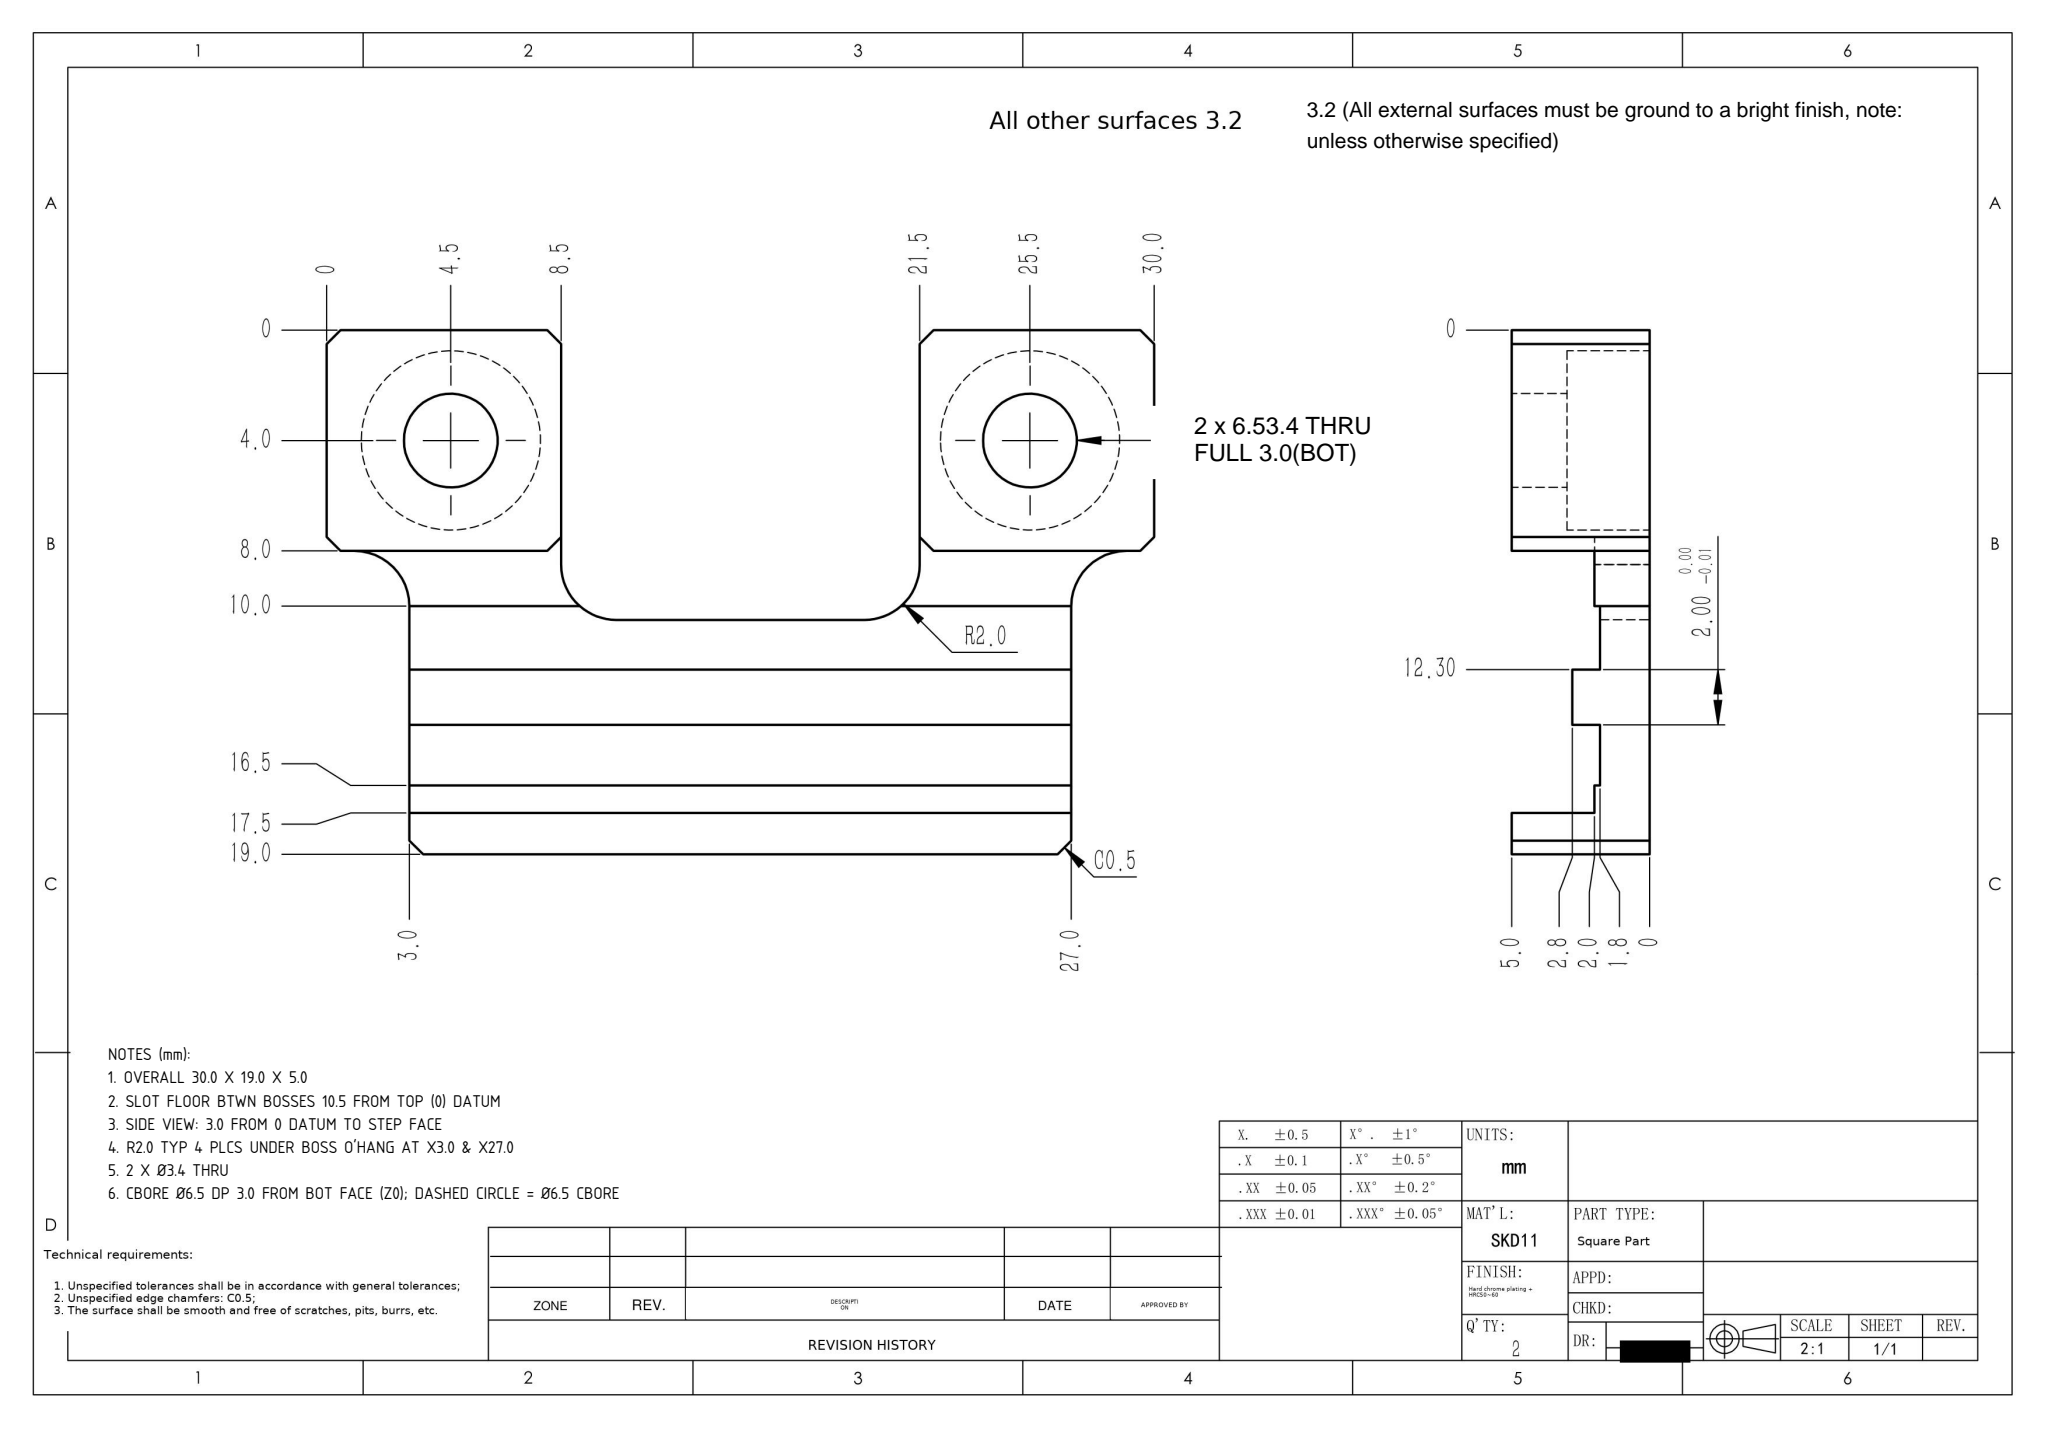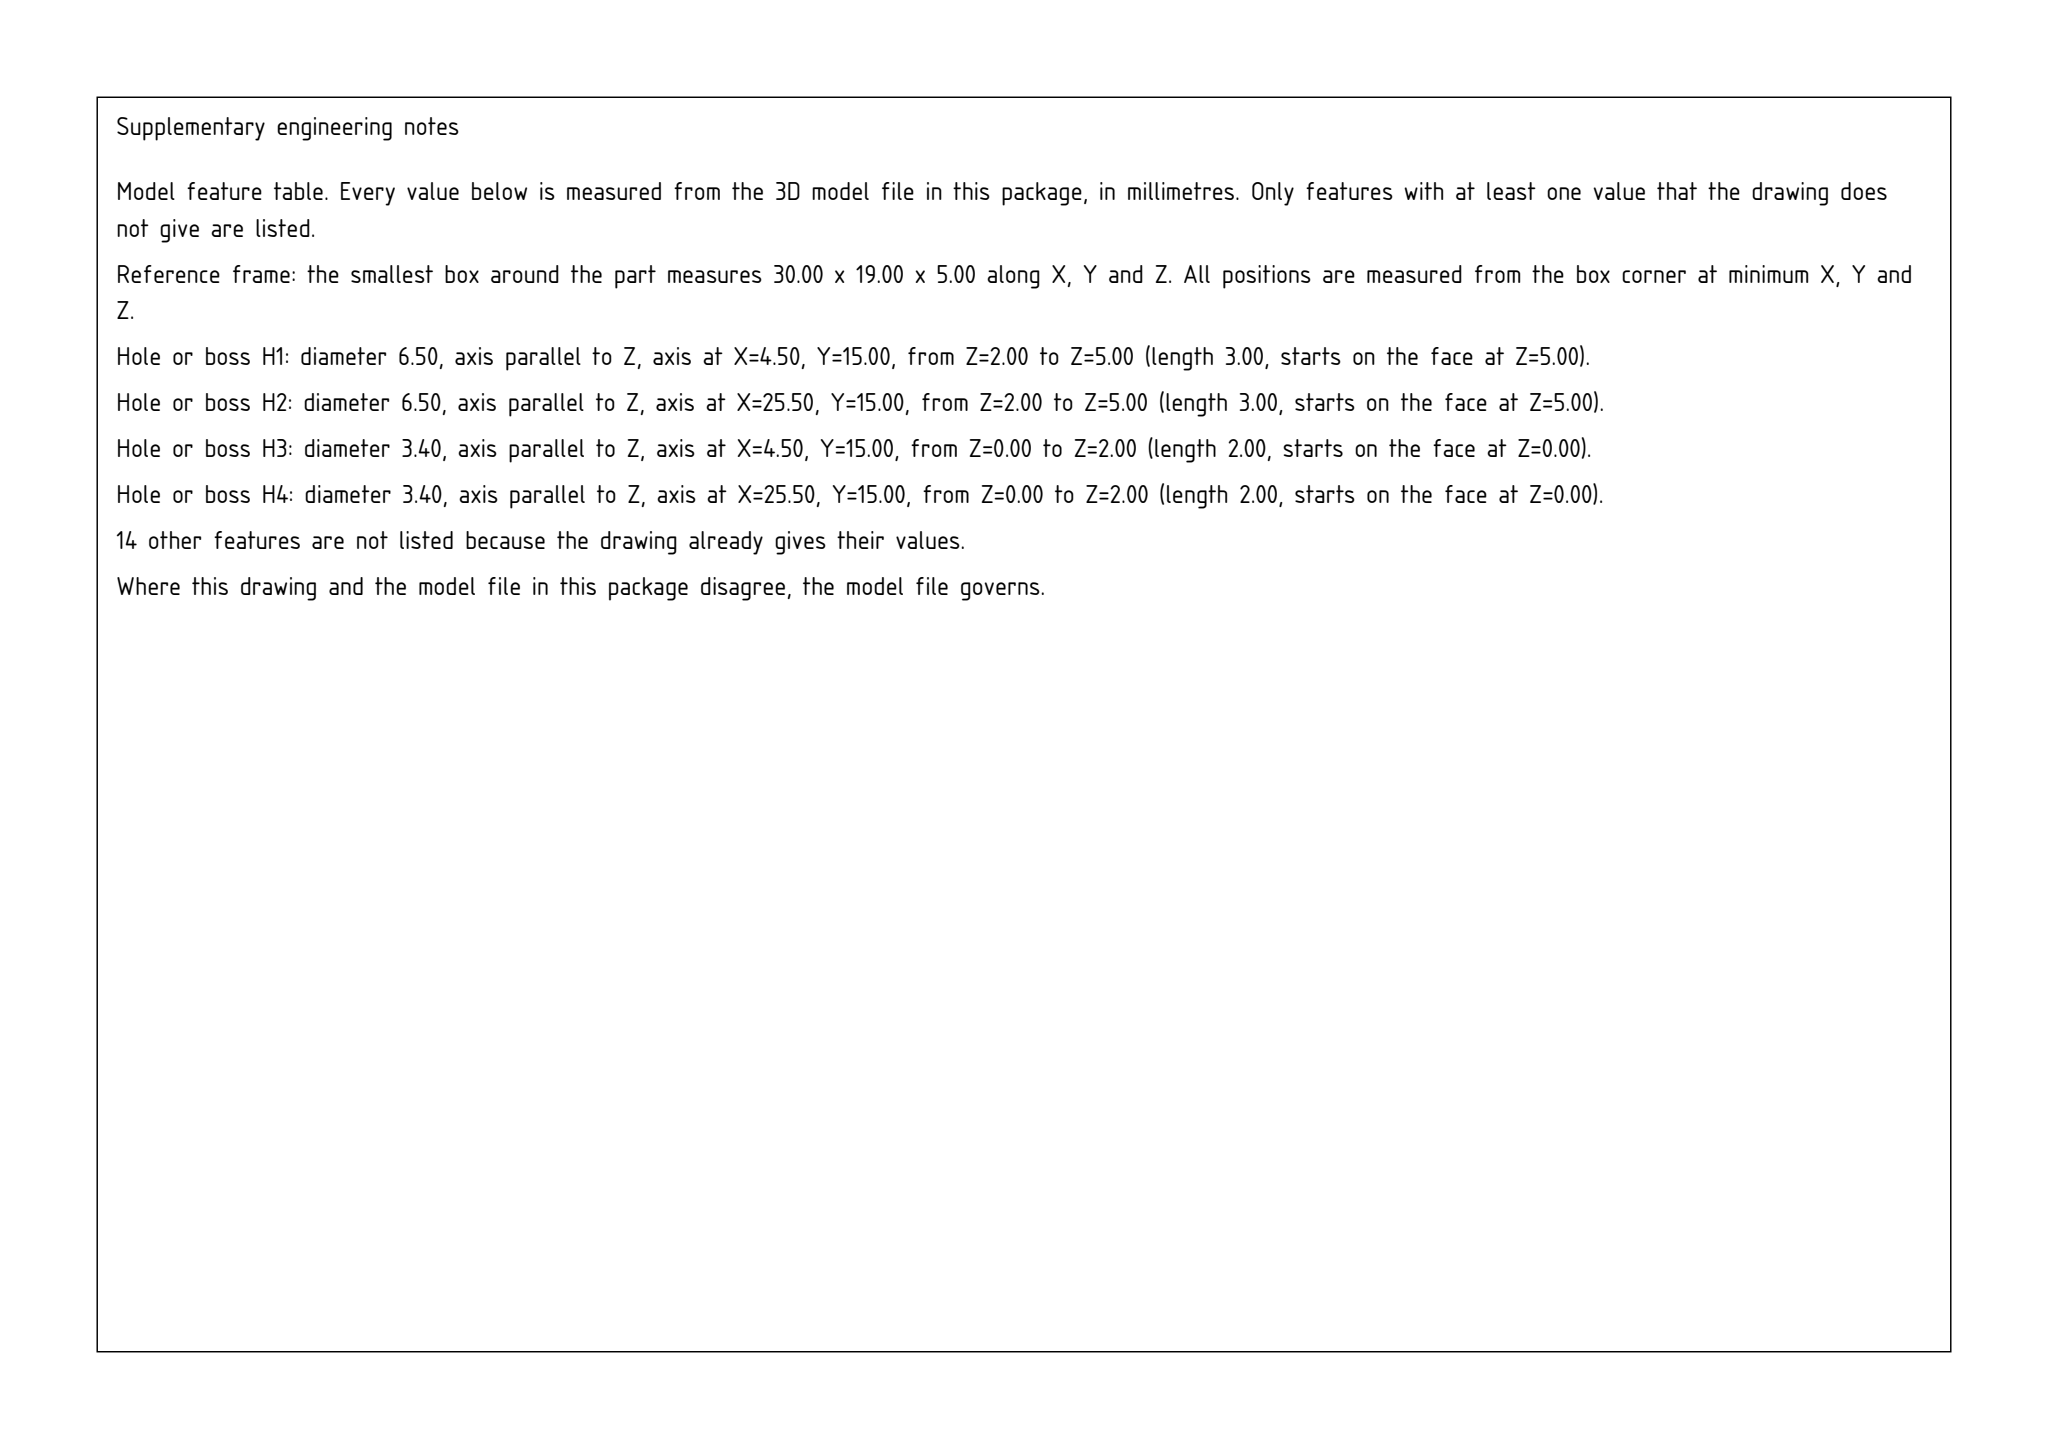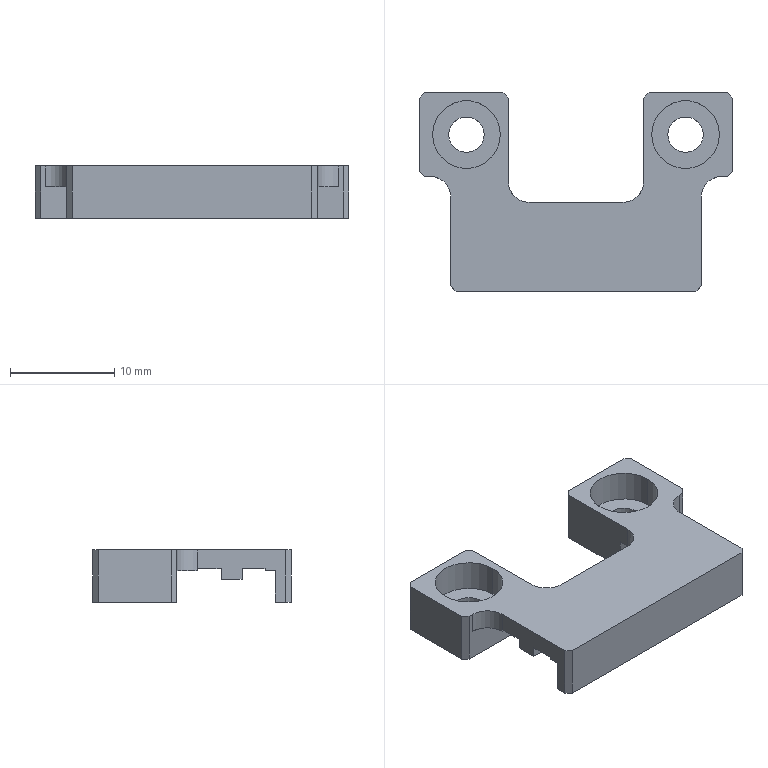Part | SolidWorks | mm | 1 solid | 52 faces | box 30 x 19 x 5 mm | volume 1035 mm3 | plane 40 | cylinder 12 | commonest cylinder face diameters 6.5 x4 3.4 x4 4 x4
Drawing notes:
OVERALL 30.0 X 19.0 X 5.0 | from the solid: bbox_xyz 30.0 x 19.0 x 5.0
SLOT FLOOR BTWN BOSSES 10.5 FROM TOP (0) DATUM | from the solid: Y-plane 8.5 in 19.0-tall bbox = 19.0-8.5 = 10.5 below top datum Y19.0
SIDE VIEW: 3.0 FROM 0 DATUM TO STEP FACE | from the solid: Z-plane 2.0 in 5.0 thk = 5.0-2.0 = 3.0 from side-view 0 datum; chain 0/1.8/2.0/2.8/5.0
R2.0 TYP 4 PLCS UNDER BOSS O'HANG AT X3.0 & X27.0 | from the solid: Ø4.0 z fillet cyls at (1.0,9.0),(29.0,9.0) tangent X3.0/X27.0 & Y11.0; inner (10.5,10.5),(19.5,10.5)
2 X Ø3.4 THRU | from the solid: cylinders dia 3.4 axis z len 2.0 at (4.5,15.0) and (25.5,15.0); 2.0+3.0=5.0 full thk
CBORE Ø6.5 DP 3.0 FROM BOT FACE (Z0); DASHED CIRCLE = Ø6.5 CBORE | from the solid: cyls dia 6.5 len 3.0 coaxial with Ø3.4 at (4.5,15.0) & (25.5,15.0); z planes 0.0 and 3.0